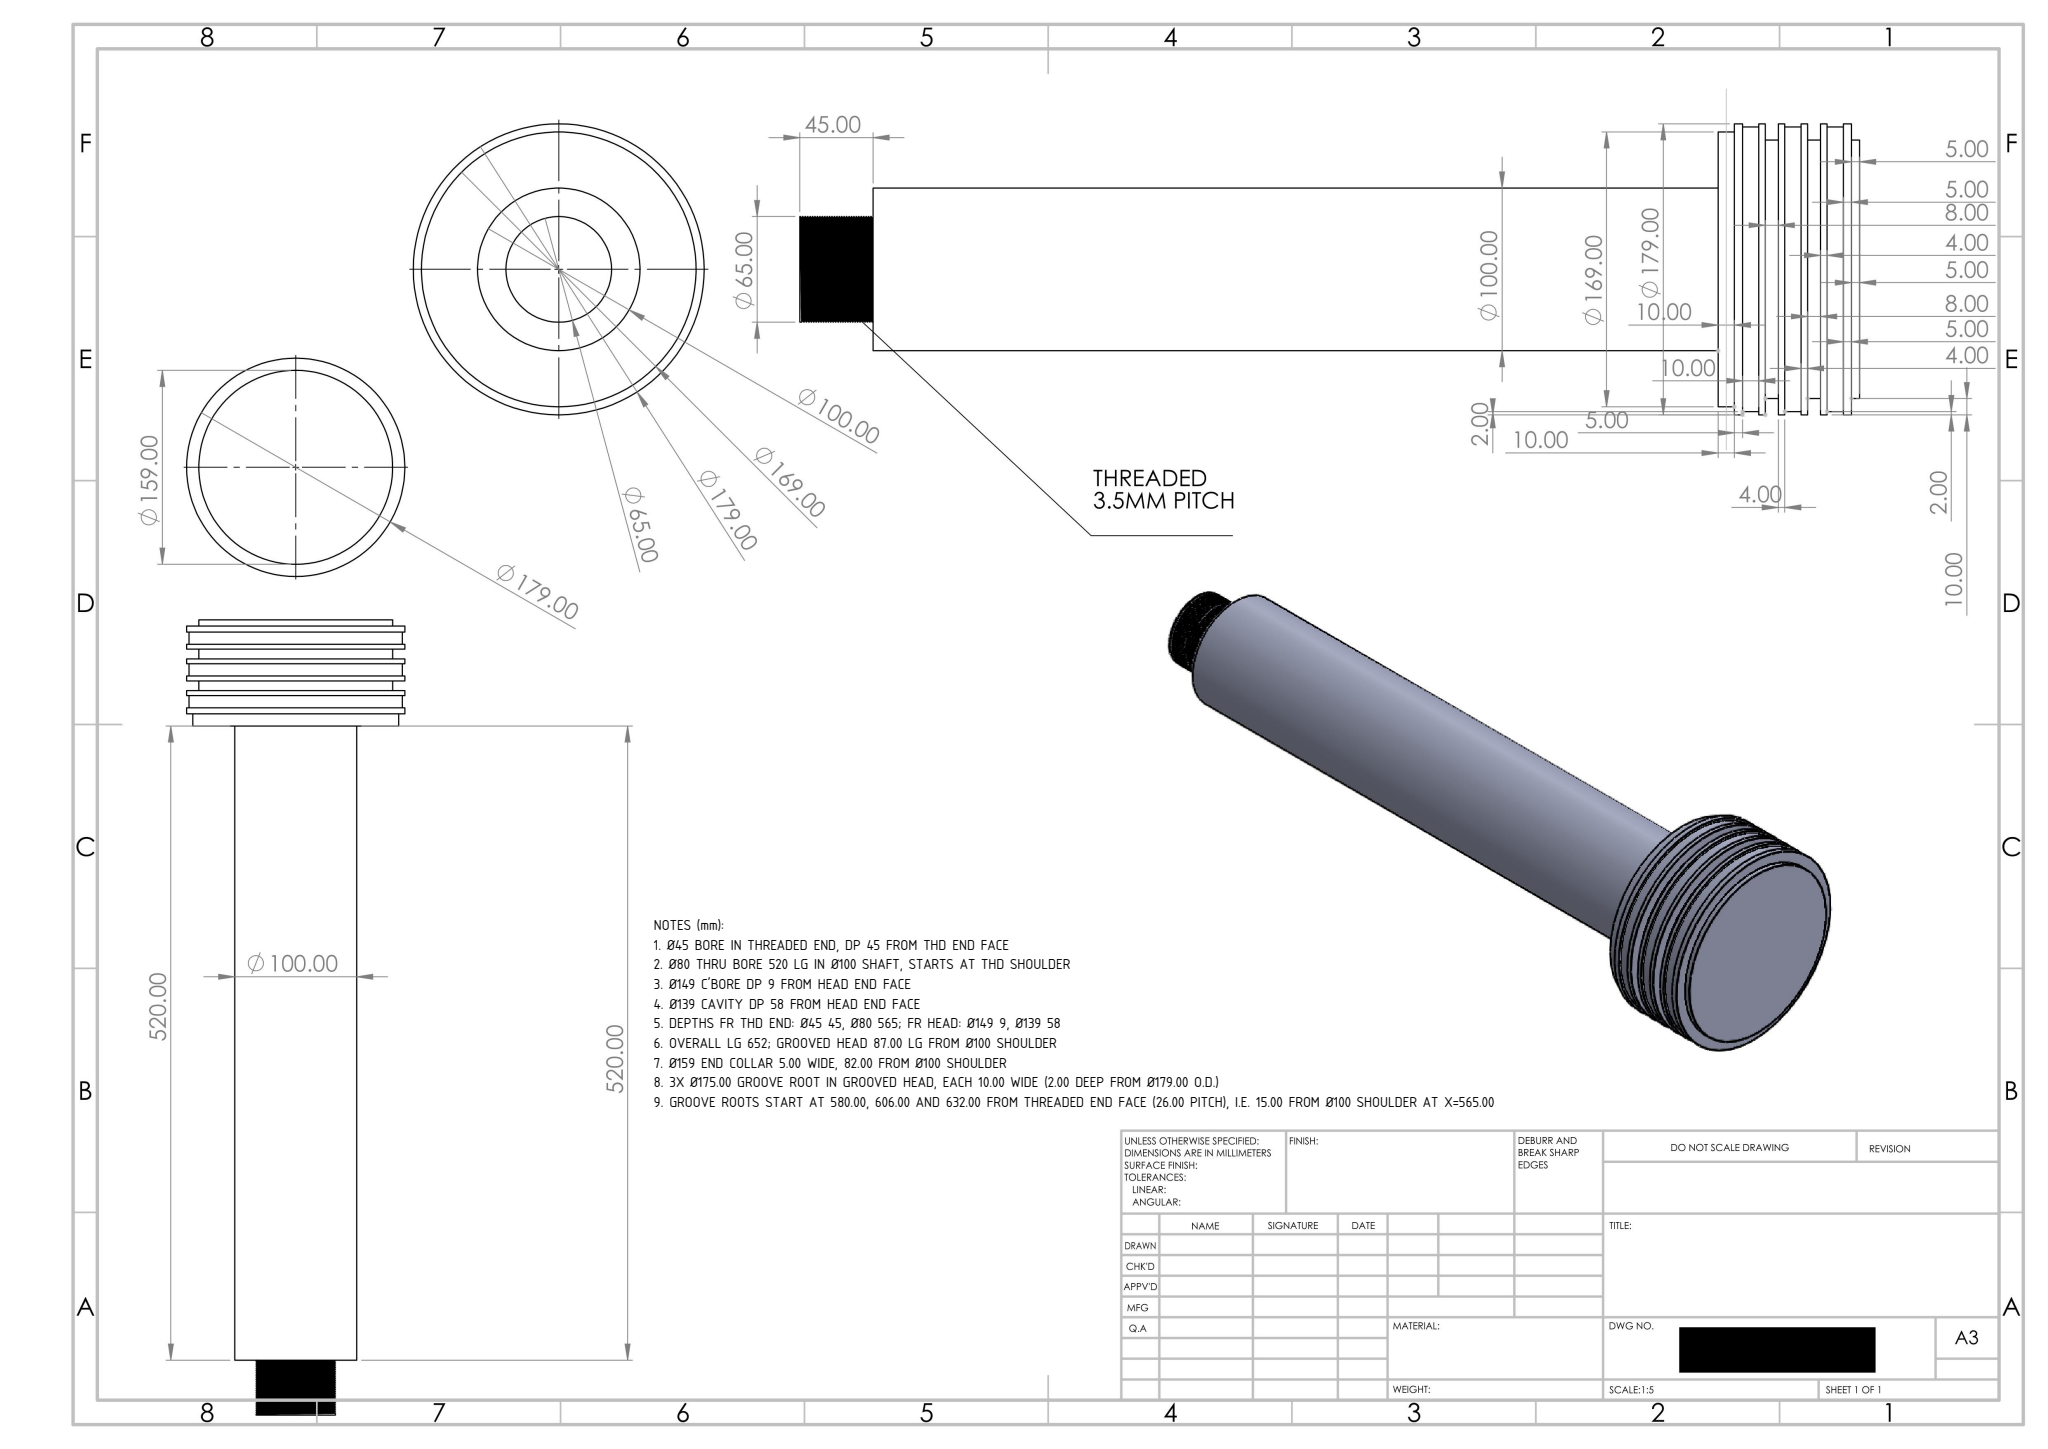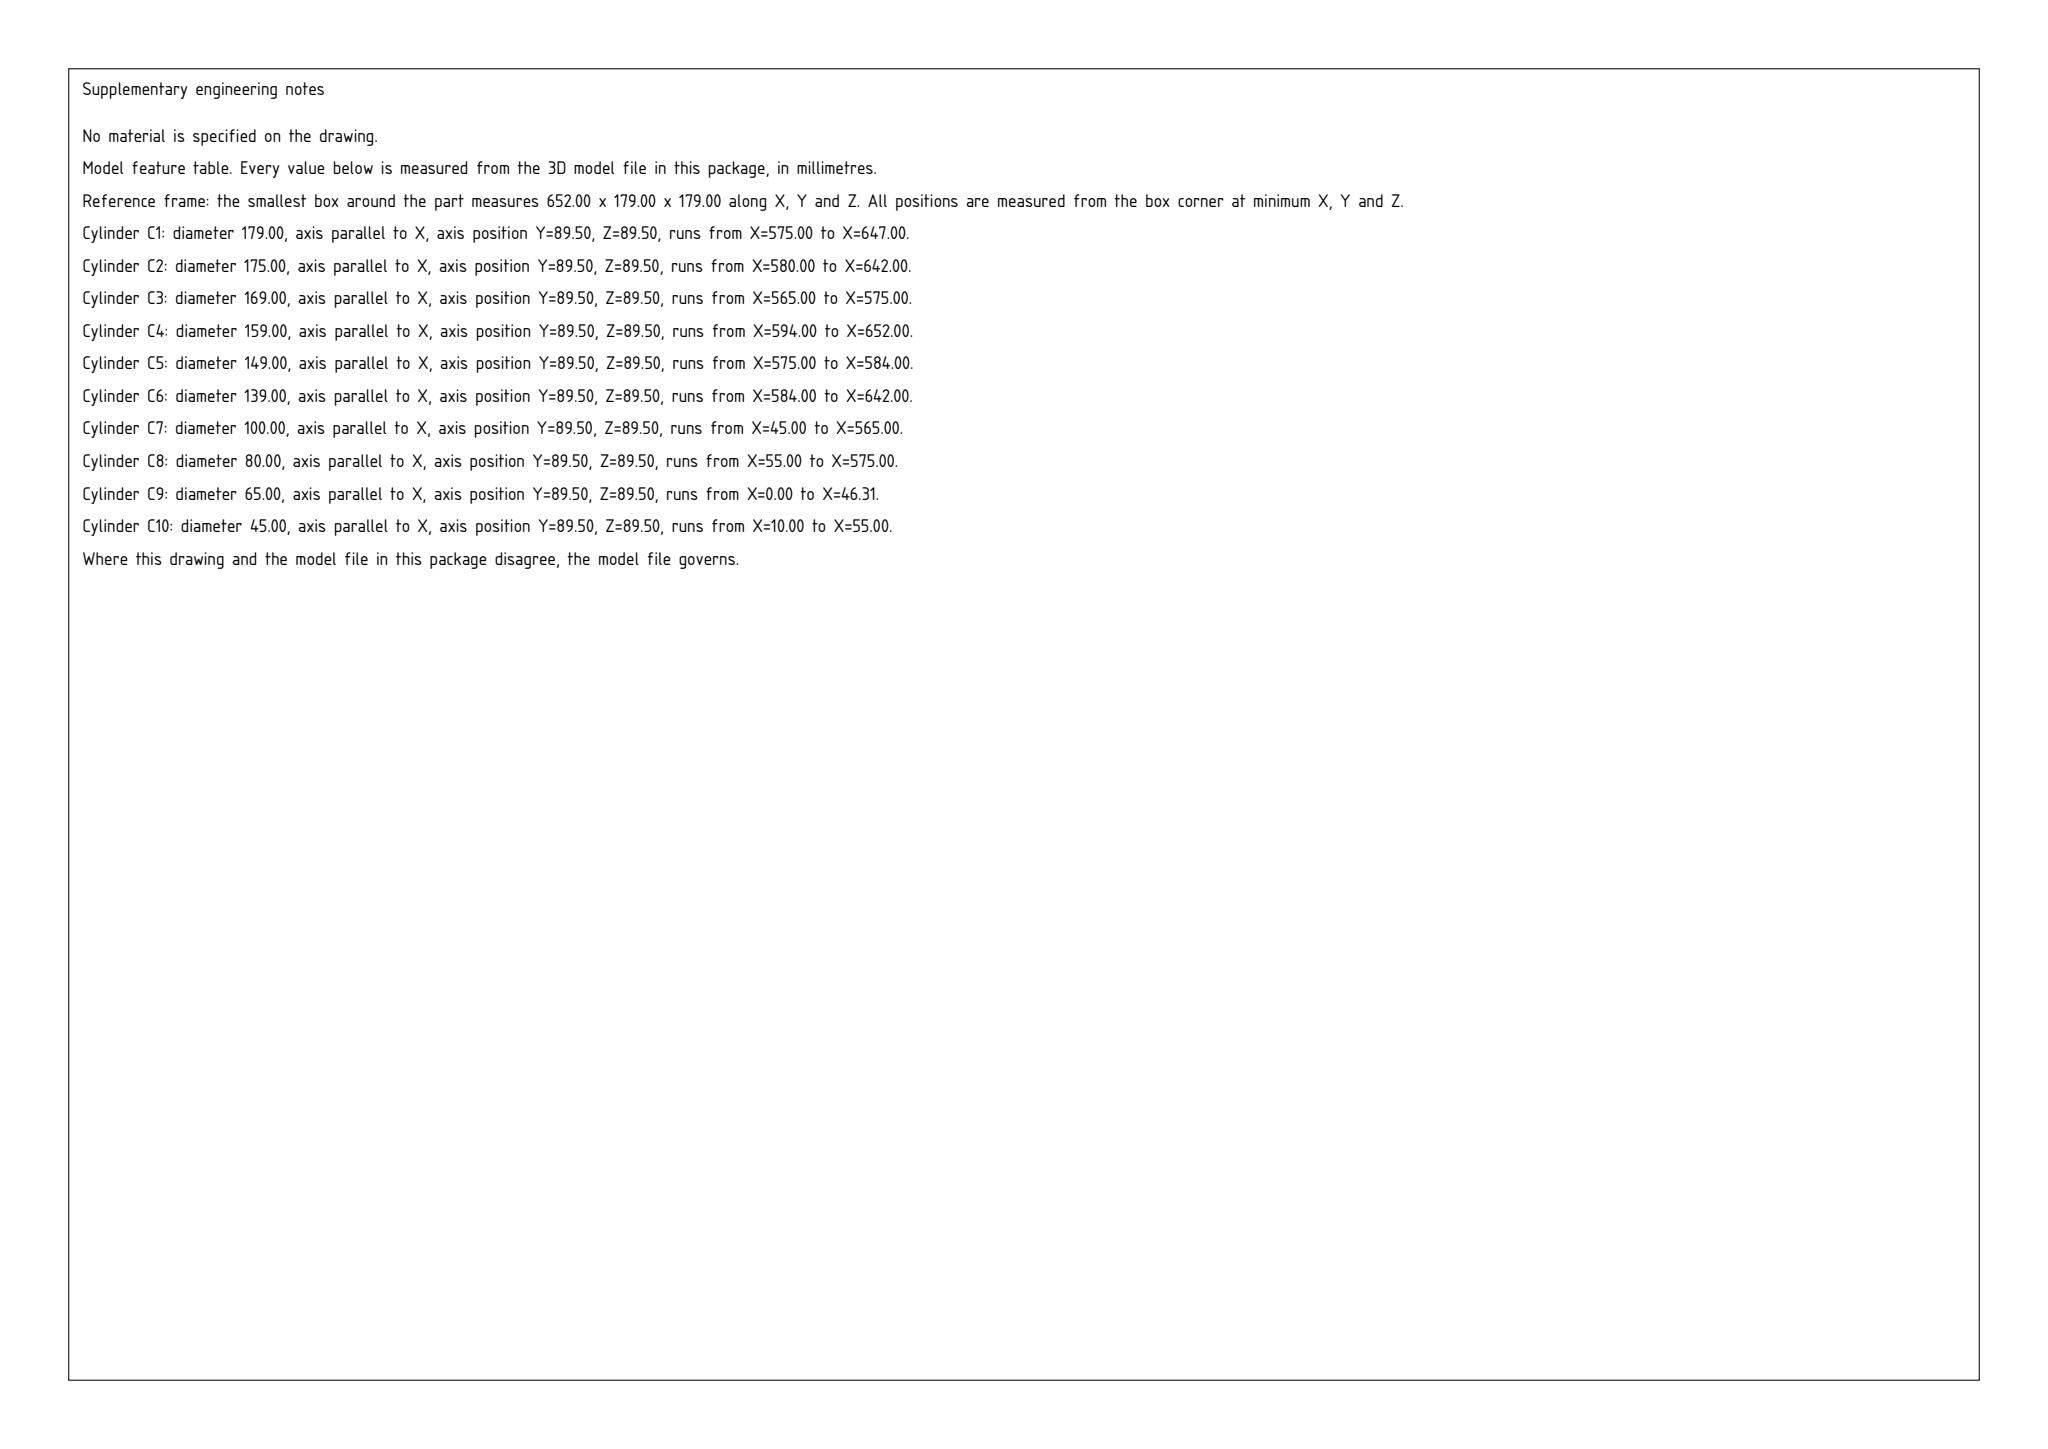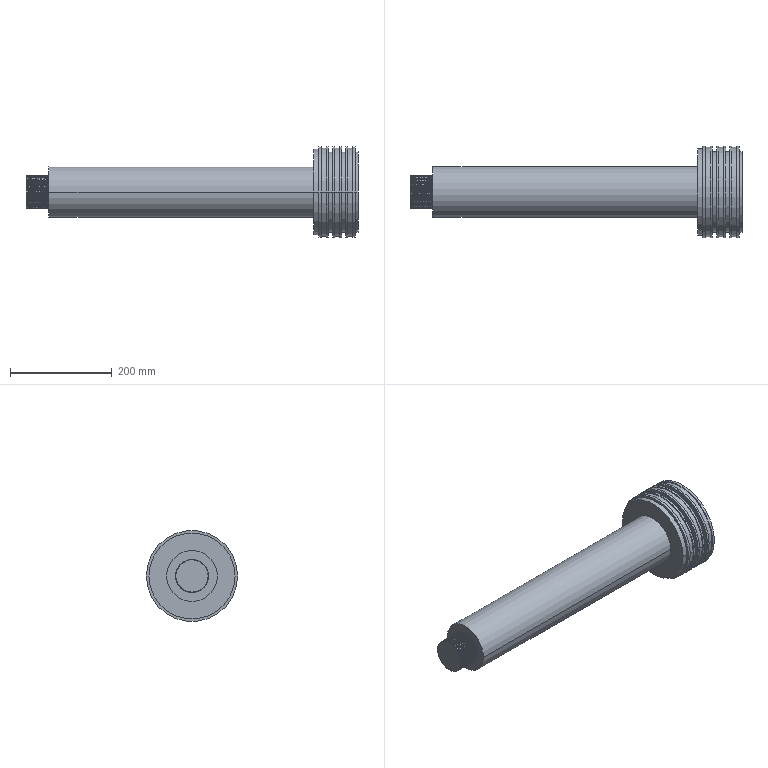Part | SolidWorks | mm | 1 solid | 126 faces | box 652 x 179 x 179 mm | volume 2523563 mm3 | cylinder 100 | plane 23 | spline 3 | commonest cylinder face diameters 65 x64 179 x12 175 x6 159 x6 100 x2 169 x2 139 x2 149 x2
Drawing notes:
Ø45 BORE IN THREADED END, DP 45 FROM THD END FACE | from the solid: cyl Ø45 x45 lg on X axis at x=0-45 (thread end face x=0)
Ø80 THRU BORE 520 LG IN Ø100 SHAFT, STARTS AT THD SHOULDER | from the solid: cyl Ø80 x520 lg, x=45 to 565; Ø100 shaft same extent
Ø149 C'BORE DP 9 FROM HEAD END FACE | from the solid: cyl Ø149 x9 lg at head end, x=643-652 (end face x=652)
Ø139 CAVITY DP 58 FROM HEAD END FACE | from the solid: cyl Ø139 x58 lg at head end, x=594-652; plane x=594
DEPTHS FR THD END: Ø45 45, Ø80 565; FR HEAD: Ø149 9, Ø139 58 | from the solid: planes x=0,45,565,594,643,652 on 652 lg part
OVERALL LG 652; GROOVED HEAD 87.00 LG FROM Ø100 SHOULDER | from the solid: bbox_xyz x=652; shaft shoulder plane x=565, head end plane x=652 (87)
Ø159 END COLLAR 5.00 WIDE, 82.00 FROM Ø100 SHOULDER | from the solid: Ø159 L=5 cyl at x=647-652; 647-565=82 from shoulder
3X Ø175.00 GROOVE ROOT IN GROOVED HEAD, EACH 10.00 WIDE (2.00 DEEP FROM Ø179.00 O.D.) | from the solid: cylinders: Ø175.00, axis x, length 10.00, count 6 (= 3 grooves, two half-faces each); Ø179.00 collar faces
GROOVE ROOTS START AT 580.00, 606.00 AND 632.00 FROM THREADED END FACE (26.00 PITCH), I.E. 15.00 FROM Ø100 SHOULDER AT X=565.00 | from the solid: axis_planes x = 580/590, 606/616, 632/642 bounding the Ø175.00 roots; x=565.00 Ø100 shoulder